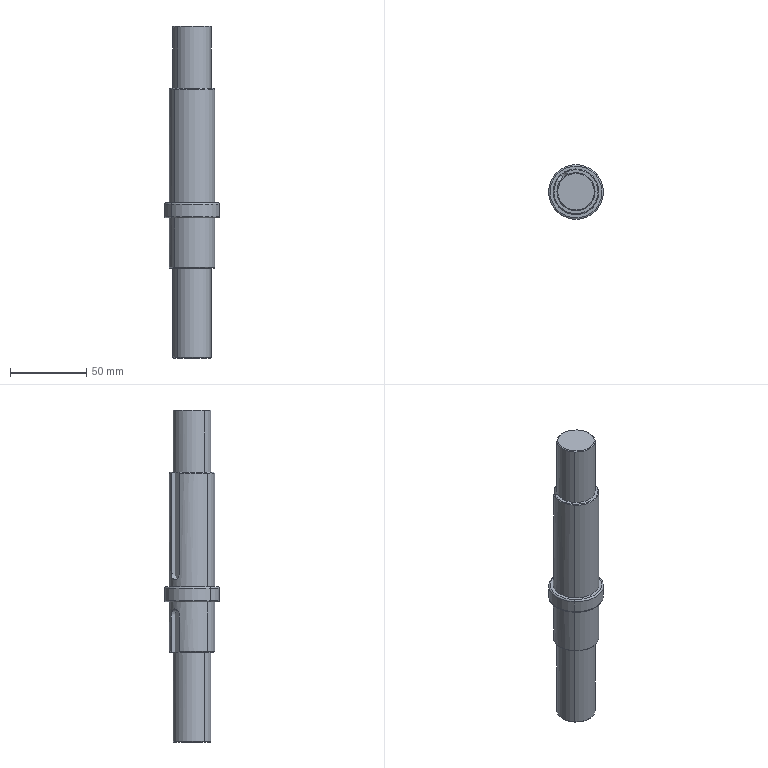Component | SolidWorks | IntermediateAxis-1 | 1 solid | 42 faces | volume 132704 mm3 | cylinder 14 | plane 14 | cone 10 | torus 4 | commonest cylinder face diameters 25 x4 30 x4 8 x4 36 x2